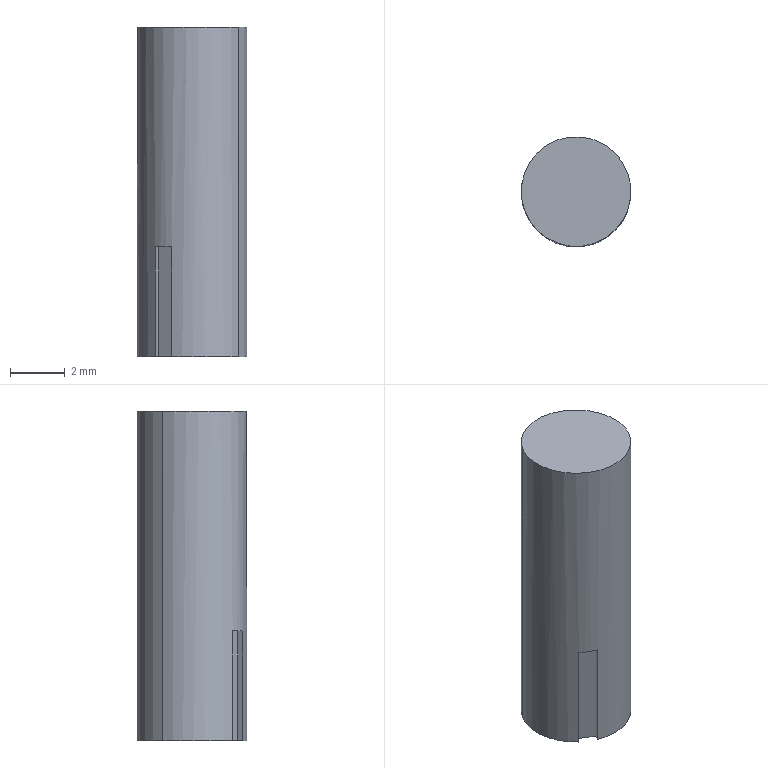Component | SolidWorks | FrontAxis-2 | 1 solid | 8 faces | box 4 x 4 x 12 mm | volume 150 mm3 | plane 6 | cylinder 2 | commonest cylinder face diameters 4 x2
build123d program:
from build123d import *

# Parameters (mm, degrees)
BOSS_EXTRUDE1_DEPTH      = 5
BOSS_EXTRUDE1_DEPTH_BACK = 7
SKETCH2_R                = 2
CUT_EXTRUDE1_START       = -3
SKETCH3_W                = 0.7
SKETCH3_H                = 0.5
CUT_EXTRUDE1_DEPTH       = 8.1


with BuildPart() as part:
    # Sketch2 → Boss-Extrude1 (new, two sides: drawn at the far end of the back side and taken through both)
    with BuildSketch(Plane.XY.offset(-BOSS_EXTRUDE1_DEPTH_BACK)):
        with Locations((-5, 0)):
            Circle(SKETCH2_R)
    extrude(amount=BOSS_EXTRUDE1_DEPTH + BOSS_EXTRUDE1_DEPTH_BACK)

    # Sketch3 → Cut-Extrude1 (cut, through all)
    with BuildSketch(Plane.XY.offset(CUT_EXTRUDE1_START)):
        with Locations((-5, 2)):
            Rectangle(SKETCH3_W, SKETCH3_H)
    extrude(amount=-CUT_EXTRUDE1_DEPTH, mode=Mode.SUBTRACT)


solid = part.part

# Placed as in the assembly
solid = solid.moved(Location((-14.243, 0.1456, 2), (0, 0, 148.053)))
STEP:
#1=COLOUR_RGB('',0.7922,0.8196,0.9333);
#2=FILL_AREA_STYLE_COLOUR('',#1);
#3=FILL_AREA_STYLE('',(#2));
#4=SURFACE_STYLE_FILL_AREA(#3);
#5=SURFACE_SIDE_STYLE('',(#4));
#6=SURFACE_STYLE_USAGE(.BOTH.,#5);
#7=PRESENTATION_STYLE_ASSIGNMENT((#6));
#8=CARTESIAN_POINT('',(-0.423,-0.1715,-0.1969));
#9=VERTEX_POINT('',#8);
#10=CARTESIAN_POINT('',(-0.3269,-0.1401,-0.1969));
#11=VERTEX_POINT('',#10);
#12=CARTESIAN_POINT('',(-0.3937,-0.09843,-0.1969));
#13=DIRECTION('',(-0.,-0.,1.));
#14=DIRECTION('',(-0.8485,0.5291,0.));
#15=AXIS2_PLACEMENT_3D('',#12,#13,#14);
#16=CIRCLE('',#15,0.07874);
#17=EDGE_CURVE('',#9,#11,#16,.T.);
#18=ORIENTED_EDGE('',*,*,#17,.T.);
#19=CARTESIAN_POINT('',(-0.3269,-0.1401,0.2756));
#20=VERTEX_POINT('',#19);
#21=CARTESIAN_POINT('',(-0.3269,-0.1401,-0.1969));
#22=DIRECTION('',(-0.,-0.,1.));
#23=VECTOR('',#22,39.37);
#24=LINE('',#21,#23);
#25=EDGE_CURVE('',#11,#20,#24,.T.);
#26=ORIENTED_EDGE('',*,*,#25,.T.);
#27=CARTESIAN_POINT('',(-0.4605,-0.05676,0.2756));
#28=VERTEX_POINT('',#27);
#29=CARTESIAN_POINT('',(-0.3937,-0.09843,0.2756));
#30=DIRECTION('',(-0.,-0.,1.));
#31=DIRECTION('',(-0.8485,0.5291,0.));
#32=AXIS2_PLACEMENT_3D('',#29,#30,#31);
#33=CIRCLE('',#32,0.07874);
#34=EDGE_CURVE('',#28,#20,#33,.T.);
#35=ORIENTED_EDGE('',*,*,#34,.F.);
#36=CARTESIAN_POINT('',(-0.4605,-0.05676,-0.1969));
#37=VERTEX_POINT('',#36);
#38=CARTESIAN_POINT('',(-0.4605,-0.05676,-0.1969));
#39=DIRECTION('',(-0.,-0.,1.));
#40=VECTOR('',#39,39.37);
#41=LINE('',#38,#40);
#42=EDGE_CURVE('',#37,#28,#41,.T.);
#43=ORIENTED_EDGE('',*,*,#42,.F.);
#44=CARTESIAN_POINT('',(-0.4464,-0.1569,-0.1969));
#45=VERTEX_POINT('',#44);
#46=CARTESIAN_POINT('',(-0.3937,-0.09843,-0.1969));
#47=DIRECTION('',(-0.,-0.,1.));
#48=DIRECTION('',(-0.8485,0.5291,0.));
#49=AXIS2_PLACEMENT_3D('',#46,#47,#48);
#50=CIRCLE('',#49,0.07874);
#51=EDGE_CURVE('',#37,#45,#50,.T.);
#52=ORIENTED_EDGE('',*,*,#51,.T.);
#53=CARTESIAN_POINT('',(-0.4464,-0.1569,-0.03937));
#54=VERTEX_POINT('',#53);
#55=CARTESIAN_POINT('',(-0.4464,-0.1569,-0.1969));
#56=DIRECTION('',(0.,0.,-1.));
#57=VECTOR('',#56,39.37);
#58=LINE('',#55,#57);
#59=EDGE_CURVE('',#54,#45,#58,.T.);
#60=ORIENTED_EDGE('',*,*,#59,.F.);
#61=CARTESIAN_POINT('',(-0.423,-0.1715,-0.03937));
#62=VERTEX_POINT('',#61);
#63=CARTESIAN_POINT('',(-0.3937,-0.09843,-0.03937));
#64=DIRECTION('',(0.,0.,-1.));
#65=DIRECTION('',(-0.8485,0.5291,0.));
#66=AXIS2_PLACEMENT_3D('',#63,#64,#65);
#67=CIRCLE('',#66,0.07874);
#68=EDGE_CURVE('',#62,#54,#67,.T.);
#69=ORIENTED_EDGE('',*,*,#68,.F.);
#70=CARTESIAN_POINT('',(-0.423,-0.1715,-0.1969));
#71=DIRECTION('',(-0.,-0.,1.));
#72=VECTOR('',#71,39.37);
#73=LINE('',#70,#72);
#74=EDGE_CURVE('',#9,#62,#73,.T.);
#75=ORIENTED_EDGE('',*,*,#74,.F.);
#76=EDGE_LOOP('',(#18,#26,#35,#43,#52,#60,#69,#75));
#77=FACE_OUTER_BOUND('',#76,.T.);
#78=CARTESIAN_POINT('',(-0.3937,-0.09843,-0.1969));
#79=DIRECTION('',(-0.,-0.,1.));
#80=DIRECTION('',(-0.8485,0.5291,0.));
#81=AXIS2_PLACEMENT_3D('',#78,#79,#80);
#82=CYLINDRICAL_SURFACE('',#81,0.07874);
#83=ADVANCED_FACE('',(#77),#82,.T.);
#84=ORIENTED_EDGE('',*,*,#25,.F.);
#85=CARTESIAN_POINT('',(-0.3937,-0.09843,-0.1969));
#86=DIRECTION('',(-0.,-0.,1.));
#87=DIRECTION('',(-0.8485,0.5291,0.));
#88=AXIS2_PLACEMENT_3D('',#85,#86,#87);
#89=CIRCLE('',#88,0.07874);
#90=EDGE_CURVE('',#11,#37,#89,.T.);
#91=ORIENTED_EDGE('',*,*,#90,.T.);
#92=ORIENTED_EDGE('',*,*,#42,.T.);
#93=CARTESIAN_POINT('',(-0.3937,-0.09843,0.2756));
#94=DIRECTION('',(-0.,-0.,1.));
#95=DIRECTION('',(-0.8485,0.5291,0.));
#96=AXIS2_PLACEMENT_3D('',#93,#94,#95);
#97=CIRCLE('',#96,0.07874);
#98=EDGE_CURVE('',#20,#28,#97,.T.);
#99=ORIENTED_EDGE('',*,*,#98,.F.);
#100=EDGE_LOOP('',(#84,#91,#92,#99));
#101=FACE_OUTER_BOUND('',#100,.T.);
#102=CARTESIAN_POINT('',(-0.3937,-0.09843,-0.1969));
#103=DIRECTION('',(-0.,-0.,1.));
#104=DIRECTION('',(-0.8485,0.5291,0.));
#105=AXIS2_PLACEMENT_3D('',#102,#103,#104);
#106=CYLINDRICAL_SURFACE('',#105,0.07874);
#107=ADVANCED_FACE('',(#101),#106,.T.);
#108=CARTESIAN_POINT('',(-0.4185,-0.1642,-0.1969));
#109=VERTEX_POINT('',#108);
#110=CARTESIAN_POINT('',(-0.4418,-0.1496,-0.1969));
#111=VERTEX_POINT('',#110);
#112=CARTESIAN_POINT('',(-0.4185,-0.1642,-0.1969));
#113=DIRECTION('',(-0.8485,0.5291,0.));
#114=VECTOR('',#113,39.37);
#115=LINE('',#112,#114);
#116=EDGE_CURVE('',#109,#111,#115,.T.);
#117=ORIENTED_EDGE('',*,*,#116,.T.);
#118=CARTESIAN_POINT('',(-0.4523,-0.1663,-0.1969));
#119=DIRECTION('',(-0.5291,-0.8485,-0.));
#120=VECTOR('',#119,39.37);
#121=LINE('',#118,#120);
#122=EDGE_CURVE('',#111,#45,#121,.T.);
#123=ORIENTED_EDGE('',*,*,#122,.T.);
#124=ORIENTED_EDGE('',*,*,#51,.F.);
#125=ORIENTED_EDGE('',*,*,#90,.F.);
#126=ORIENTED_EDGE('',*,*,#17,.F.);
#127=CARTESIAN_POINT('',(-0.382,-0.1057,-0.1969));
#128=DIRECTION('',(0.5291,0.8485,0.));
#129=VECTOR('',#128,39.37);
#130=LINE('',#127,#129);
#131=EDGE_CURVE('',#9,#109,#130,.T.);
#132=ORIENTED_EDGE('',*,*,#131,.T.);
#133=EDGE_LOOP('',(#117,#123,#124,#125,#126,#132));
#134=FACE_OUTER_BOUND('',#133,.T.);
#135=CARTESIAN_POINT('',(-0.3937,-0.09843,-0.1969));
#136=DIRECTION('',(-0.,-0.,1.));
#137=DIRECTION('',(-0.8485,0.5291,0.));
#138=AXIS2_PLACEMENT_3D('',#135,#136,#137);
#139=PLANE('',#138);
#140=ADVANCED_FACE('',(#134),#139,.F.);
#141=ORIENTED_EDGE('',*,*,#34,.T.);
#142=ORIENTED_EDGE('',*,*,#98,.T.);
#143=EDGE_LOOP('',(#141,#142));
#144=FACE_OUTER_BOUND('',#143,.T.);
#145=CARTESIAN_POINT('',(-0.3937,-0.09843,0.2756));
#146=DIRECTION('',(-0.,-0.,1.));
#147=DIRECTION('',(-0.8485,0.5291,0.));
#148=AXIS2_PLACEMENT_3D('',#145,#146,#147);
#149=PLANE('',#148);
#150=ADVANCED_FACE('',(#144),#149,.T.);
#151=ORIENTED_EDGE('',*,*,#59,.T.);
#152=ORIENTED_EDGE('',*,*,#122,.F.);
#153=CARTESIAN_POINT('',(-0.4418,-0.1496,-0.03937));
#154=VERTEX_POINT('',#153);
#155=CARTESIAN_POINT('',(-0.4418,-0.1496,-0.1969));
#156=DIRECTION('',(-0.,-0.,1.));
#157=VECTOR('',#156,39.37);
#158=LINE('',#155,#157);
#159=EDGE_CURVE('',#111,#154,#158,.T.);
#160=ORIENTED_EDGE('',*,*,#159,.T.);
#161=CARTESIAN_POINT('',(-0.4523,-0.1663,-0.03937));
#162=DIRECTION('',(-0.5291,-0.8485,-0.));
#163=VECTOR('',#162,39.37);
#164=LINE('',#161,#163);
#165=EDGE_CURVE('',#154,#54,#164,.T.);
#166=ORIENTED_EDGE('',*,*,#165,.T.);
#167=EDGE_LOOP('',(#151,#152,#160,#166));
#168=FACE_OUTER_BOUND('',#167,.T.);
#169=CARTESIAN_POINT('',(-0.4523,-0.1663,-0.1969));
#170=DIRECTION('',(-0.8485,0.5291,0.));
#171=DIRECTION('',(0.,0.,-1.));
#172=AXIS2_PLACEMENT_3D('',#169,#170,#171);
#173=PLANE('',#172);
#174=ADVANCED_FACE('',(#168),#173,.F.);
#175=CARTESIAN_POINT('',(-0.4185,-0.1642,-0.03937));
#176=VERTEX_POINT('',#175);
#177=CARTESIAN_POINT('',(-0.4185,-0.1642,-0.03937));
#178=DIRECTION('',(-0.8485,0.5291,0.));
#179=VECTOR('',#178,39.37);
#180=LINE('',#177,#179);
#181=EDGE_CURVE('',#176,#154,#180,.T.);
#182=ORIENTED_EDGE('',*,*,#181,.T.);
#183=ORIENTED_EDGE('',*,*,#159,.F.);
#184=ORIENTED_EDGE('',*,*,#116,.F.);
#185=CARTESIAN_POINT('',(-0.4185,-0.1642,-0.1969));
#186=DIRECTION('',(-0.,-0.,1.));
#187=VECTOR('',#186,39.37);
#188=LINE('',#185,#187);
#189=EDGE_CURVE('',#109,#176,#188,.T.);
#190=ORIENTED_EDGE('',*,*,#189,.T.);
#191=EDGE_LOOP('',(#182,#183,#184,#190));
#192=FACE_OUTER_BOUND('',#191,.T.);
#193=CARTESIAN_POINT('',(-0.4185,-0.1642,-0.1969));
#194=DIRECTION('',(0.5291,0.8485,0.));
#195=DIRECTION('',(0.,0.,-1.));
#196=AXIS2_PLACEMENT_3D('',#193,#194,#195);
#197=PLANE('',#196);
#198=ADVANCED_FACE('',(#192),#197,.F.);
#199=ORIENTED_EDGE('',*,*,#74,.T.);
#200=CARTESIAN_POINT('',(-0.4289,-0.1809,-0.03937));
#201=DIRECTION('',(0.5291,0.8485,0.));
#202=VECTOR('',#201,39.37);
#203=LINE('',#200,#202);
#204=EDGE_CURVE('',#62,#176,#203,.T.);
#205=ORIENTED_EDGE('',*,*,#204,.T.);
#206=ORIENTED_EDGE('',*,*,#189,.F.);
#207=ORIENTED_EDGE('',*,*,#131,.F.);
#208=EDGE_LOOP('',(#199,#205,#206,#207));
#209=FACE_OUTER_BOUND('',#208,.T.);
#210=CARTESIAN_POINT('',(-0.4289,-0.1809,-0.1969));
#211=DIRECTION('',(0.8485,-0.5291,-0.));
#212=DIRECTION('',(-0.,-0.,1.));
#213=AXIS2_PLACEMENT_3D('',#210,#211,#212);
#214=PLANE('',#213);
#215=ADVANCED_FACE('',(#209),#214,.F.);
#216=ORIENTED_EDGE('',*,*,#68,.T.);
#217=ORIENTED_EDGE('',*,*,#165,.F.);
#218=ORIENTED_EDGE('',*,*,#181,.F.);
#219=ORIENTED_EDGE('',*,*,#204,.F.);
#220=EDGE_LOOP('',(#216,#217,#218,#219));
#221=FACE_OUTER_BOUND('',#220,.T.);
#222=CARTESIAN_POINT('',(-0.5607,0.005734,-0.03937));
#223=DIRECTION('',(-0.,-0.,1.));
#224=DIRECTION('',(-0.8485,0.5291,0.));
#225=AXIS2_PLACEMENT_3D('',#222,#223,#224);
#226=PLANE('',#225);
#227=ADVANCED_FACE('',(#221),#226,.F.);
#228=CLOSED_SHELL('',(#83,#107,#140,#150,#174,#198,#215,#227));
#229=MANIFOLD_SOLID_BREP('',#228);
#230=STYLED_ITEM('',(#7),#229);
#231=PRESENTATION_LAYER_ASSIGNMENT('','',(#230));
#232=(LENGTH_UNIT()NAMED_UNIT(*)SI_UNIT($,.METRE.));
#233=LENGTH_MEASURE_WITH_UNIT(LENGTH_MEASURE(0.0254),#232);
#234=DIMENSIONAL_EXPONENTS(1.,0.,0.,0.,0.,0.,0.);
#235=(CONVERSION_BASED_UNIT('',#233)LENGTH_UNIT()NAMED_UNIT(#234));
#236=UNCERTAINTY_MEASURE_WITH_UNIT(LENGTH_MEASURE(0.00001),#235,'','');
#237=(NAMED_UNIT(*)PLANE_ANGLE_UNIT()SI_UNIT($,.RADIAN.));
#238=(NAMED_UNIT(*)SI_UNIT($,.STERADIAN.)SOLID_ANGLE_UNIT());
#239=(GEOMETRIC_REPRESENTATION_CONTEXT(3)GLOBAL_UNCERTAINTY_ASSIGNED_CONTEXT((#236))GLOBAL_UNIT_ASSIGNED_CONTEXT((#235,#237,#238))REPRESENTATION_CONTEXT('',''));
#240=MECHANICAL_DESIGN_GEOMETRIC_PRESENTATION_REPRESENTATION('',(#230),#239);
#241=CARTESIAN_POINT('',(0.,0.,0.));
#242=DIRECTION('',(0.,0.,1.));
#243=DIRECTION('',(1.,0.,0.));
#244=AXIS2_PLACEMENT_3D('',#241,#242,#243);
#245=(LENGTH_UNIT()NAMED_UNIT(*)SI_UNIT($,.METRE.));
#246=LENGTH_MEASURE_WITH_UNIT(LENGTH_MEASURE(0.0254),#245);
#247=DIMENSIONAL_EXPONENTS(1.,0.,0.,0.,0.,0.,0.);
#248=(CONVERSION_BASED_UNIT('',#246)LENGTH_UNIT()NAMED_UNIT(#247));
#249=UNCERTAINTY_MEASURE_WITH_UNIT(LENGTH_MEASURE(0.00001),#248,'','');
#250=(NAMED_UNIT(*)PLANE_ANGLE_UNIT()SI_UNIT($,.RADIAN.));
#251=(NAMED_UNIT(*)SI_UNIT($,.STERADIAN.)SOLID_ANGLE_UNIT());
#252=(GEOMETRIC_REPRESENTATION_CONTEXT(3)GLOBAL_UNCERTAINTY_ASSIGNED_CONTEXT((#249))GLOBAL_UNIT_ASSIGNED_CONTEXT((#248,#250,#251))REPRESENTATION_CONTEXT('',''));
#253=ADVANCED_BREP_SHAPE_REPRESENTATION('',(#229,#244),#252);